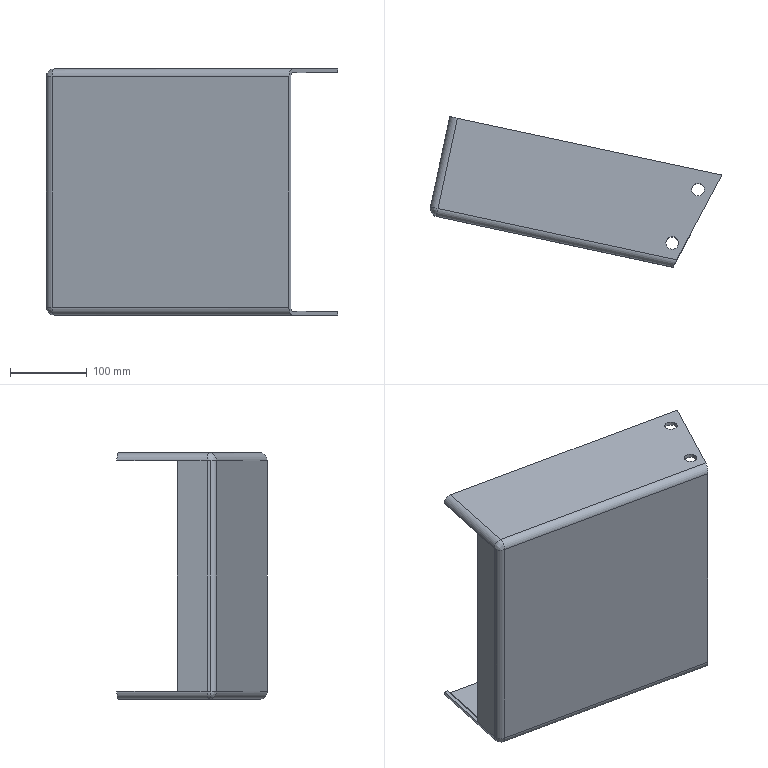Component | SolidWorks | FeedInlet-1 | 1 solid | 40 faces | volume 998955 mm3 | cylinder 20 | plane 14 | spline 6 | commonest cylinder face diameters 16.427 x8 10 x6 20 x6